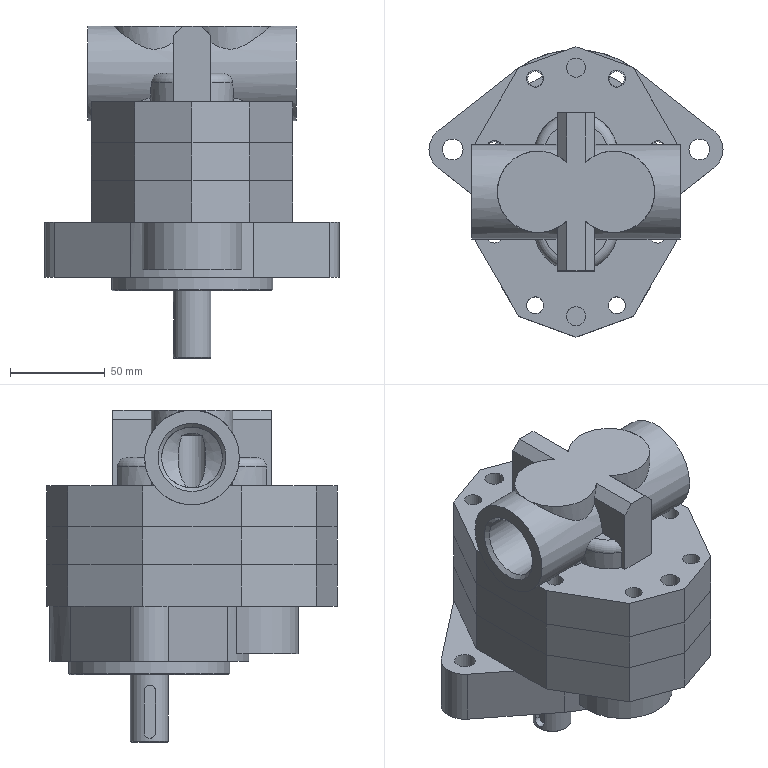Assembly | NX | mm | 8 component files | 8 solids | 406 faces | box 155 x 153 x 175 mm | volume 1244752 mm3 | plane 144 | cylinder 136 | spline 72 | cone 28 | other 22 | torus 4 | commonest cylinder face diameters 9 x24 25 x10 10 x9 15 x9 43 x8 55.5 x8 50.5 x6 4 x6
Bill of materials:
unnamed part 1 | 1 |  | Thick flat plate with a polygonal (roughly ten-sided, elongated) outline, a ring of small through holes near the edge, and a large central through opening shaped like two overlapping circles with small semicircular side lobes at the waist.
unnamed part 2 | 1 |  | Complex body on a polygonal flanged base with edge holes. A horizontal cylindrical barrel runs across the top, with a round bore at one end. Two overlapping circular disc-shaped raised faces and a central rectangular rib sit over the barrel, and rounded bosses and recesses sit between the barrel and the base.
unnamed part 3 | 1 |  | Round flange with a raised cylindrical hub on one side and a central through bore. The hub face has concentric annular recesses and curved arc slots, and the flange has three small through holes.
unnamed part 4 | 1 |  | Spur gear with nine teeth and integral cylindrical shaft stubs of similar length on both sides. Each stub has a reduced-diameter neck next to the gear face.
unnamed part 5 | 1 |  | Thick plate with an irregular outline that combines the polygonal pattern with side lugs. It has a ring of small through holes, one large through bore, one large blind bore with a conical bottom, and an elliptical groove on the top face. Cylindrical projections stand out on the underside.
unnamed part 6 | 2 |  | Thin flat figure-eight plate with two round through holes, two semicircular notches at the waist, and small notches on the outer perimeter.
unnamed part 7 | 1 |  | Spur gear with nine teeth on a shaft. There is a short journal on one side, and a longer shaft on the other side that steps down to a smaller-diameter end section.
Mates:
1. fix | CYCH_1_RearPumpCover 1 component
2. touch align | CLYB_02_PumpBody 1 face | CYCH_1_RearPumpCover 1 face
3. touch align | CLYB_02_PumpBody 1 face | CYCH_1_RearPumpCover 1 face
4. touch align | CLYB_04_FrontPumpCover 1 face | CLYB_02_PumpBody 1 face
5. touch align | CLYB_04_FrontPumpCover 1 face | CYCH_1_RearPumpCover 1 face
6. touch align | CLYB_05_CoverPlate 1 face | CLYB_04_FrontPumpCover 1 face
7. touch align | CLYB_03_WearPlate 2 face | CYCH_1_RearPumpCover 1 face
8. touch align | CLYB_03_WearPlate 2 face | CYCH_1_RearPumpCover 1 face
9. touch align | CYCH_1_RearPumpCover 1 face | CLYB_03_WearPlate 2 face
10. touch align | CLYB_02_PumpBody 1 face | CYCH_1_RearPumpCover 1 face
11. touch align | CLYB_03_WearPlate 1 face | CYCH_1_RearPumpCover 1 face
12. touch align | CLYB_03_WearPlate 1 face | CYCH_1_RearPumpCover 1 face
13. touch align | CLYB_03_WearPlate 1 face | CLYB_02_PumpBody 1 face
14. touch align | CLYB_04_FrontPumpCover 1 face | CLYB_02_PumpBody 1 face
15. touch align | CLYB_05_CoverPlate 1 face | CLYB_04_FrontPumpCover 1 face
16. touch align | CLYB_07_OutputGearShaft 1 face | CLYB_04_FrontPumpCover 1 face
17. touch align | CLYB_07_OutputGearShaft 1 face | CLYB_03_WearPlate 1 face
18. touch align | CLYB_07_InputGearShaft 1 face | CLYB_04_FrontPumpCover 1 face
19. touch align | CLYB_03_WearPlate 1 face | CLYB_07_InputGearShaft 1 face
20. touch align | CLYB_07_OutputGearShaft 1 face | CLYB_07_InputGearShaft 1 face